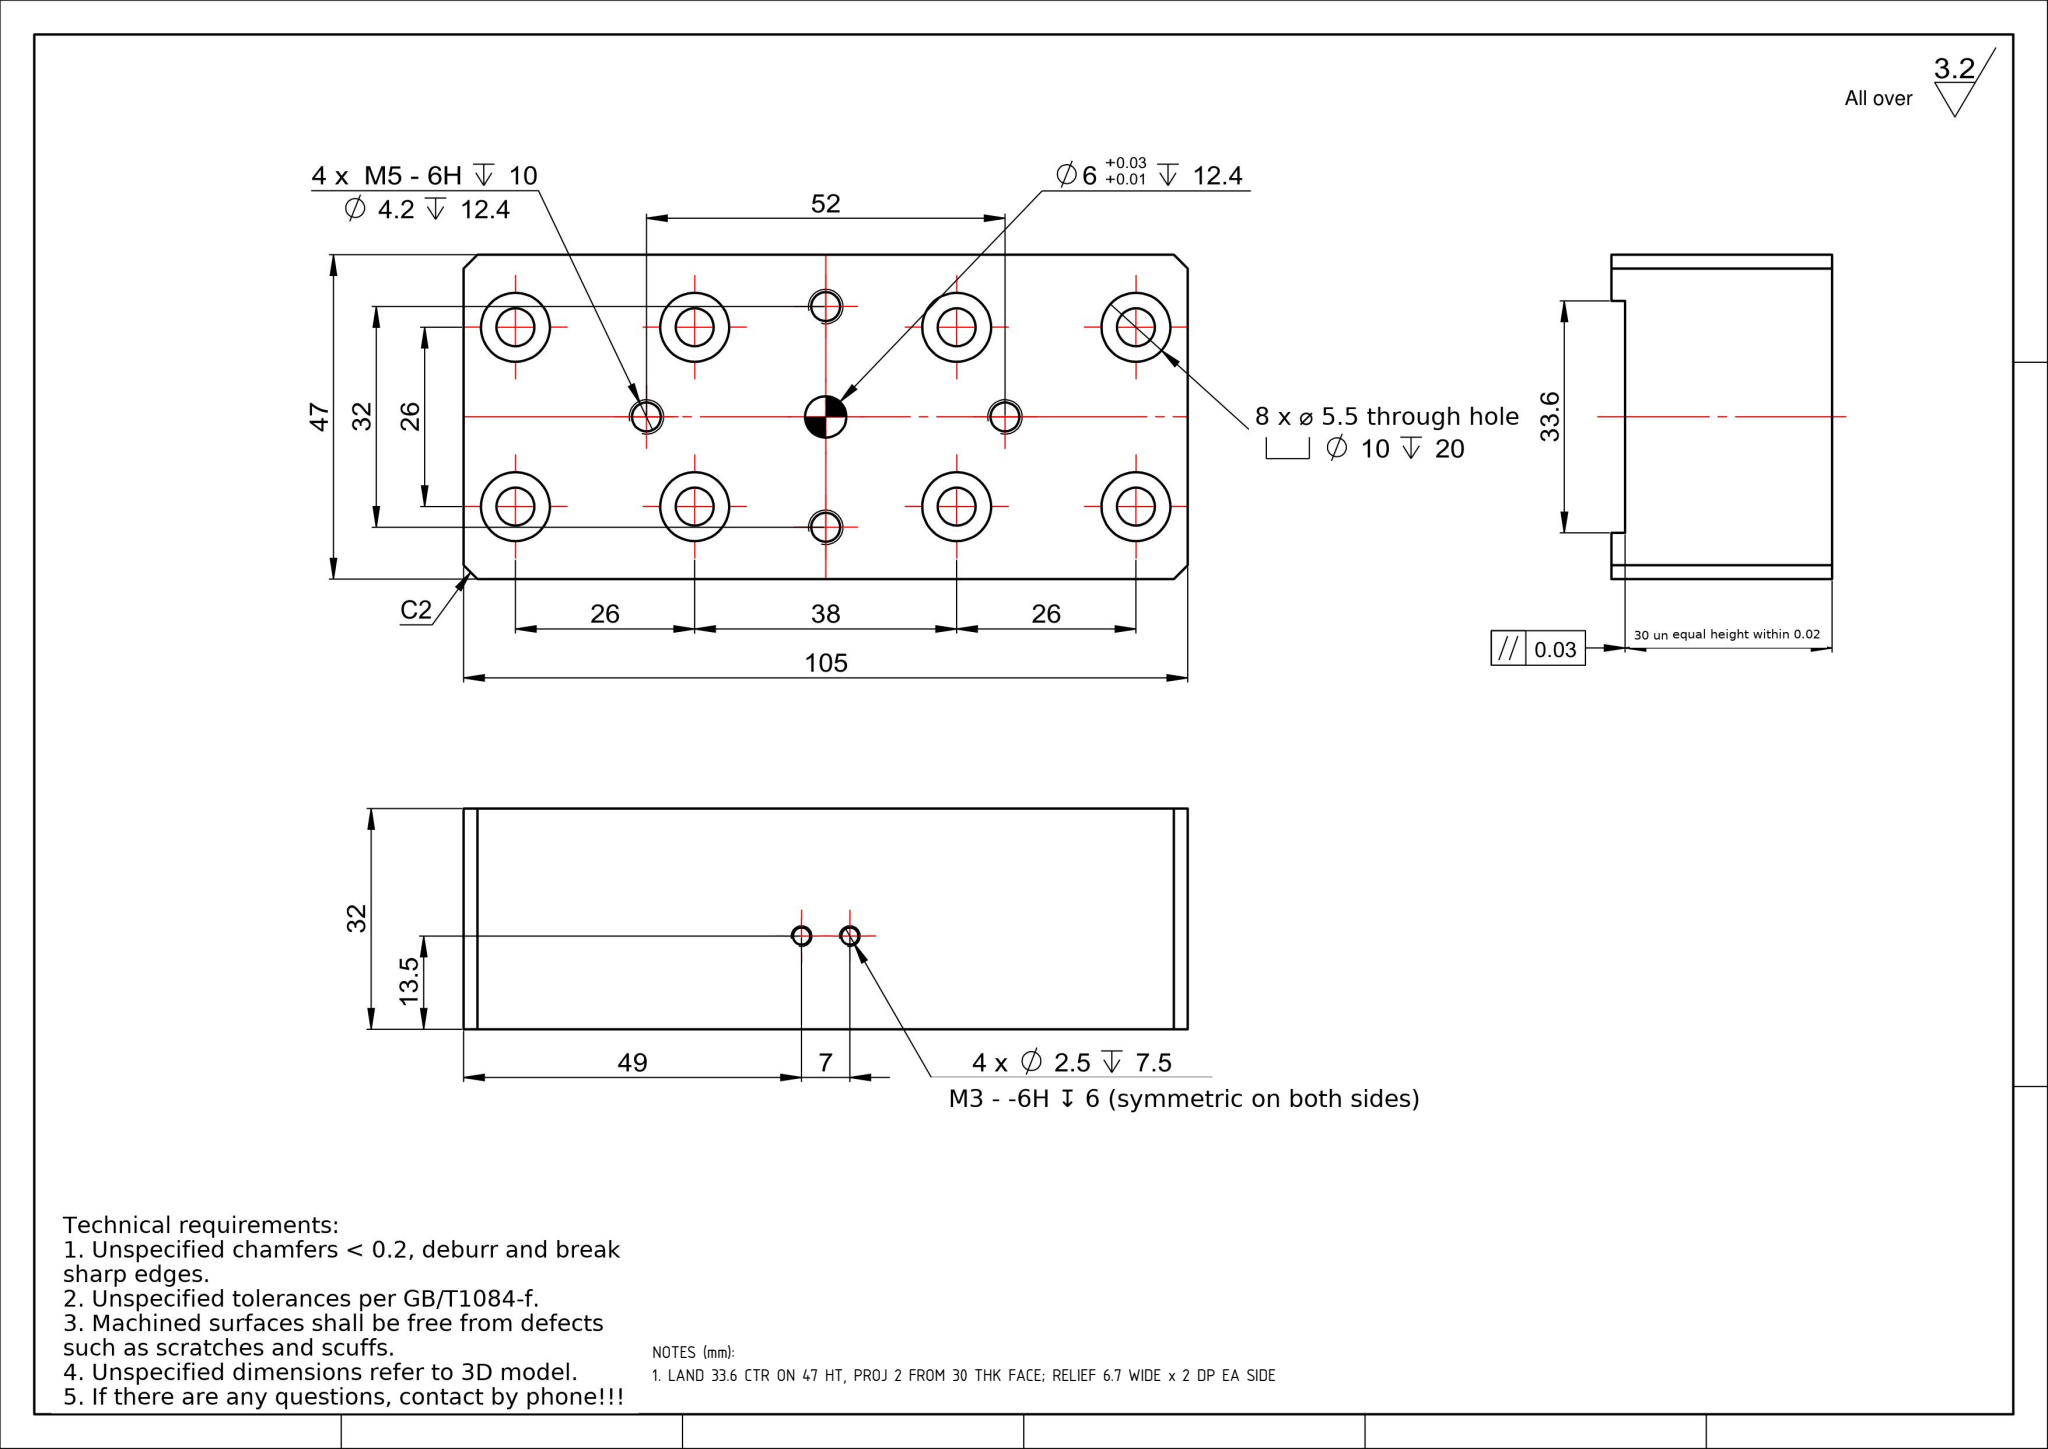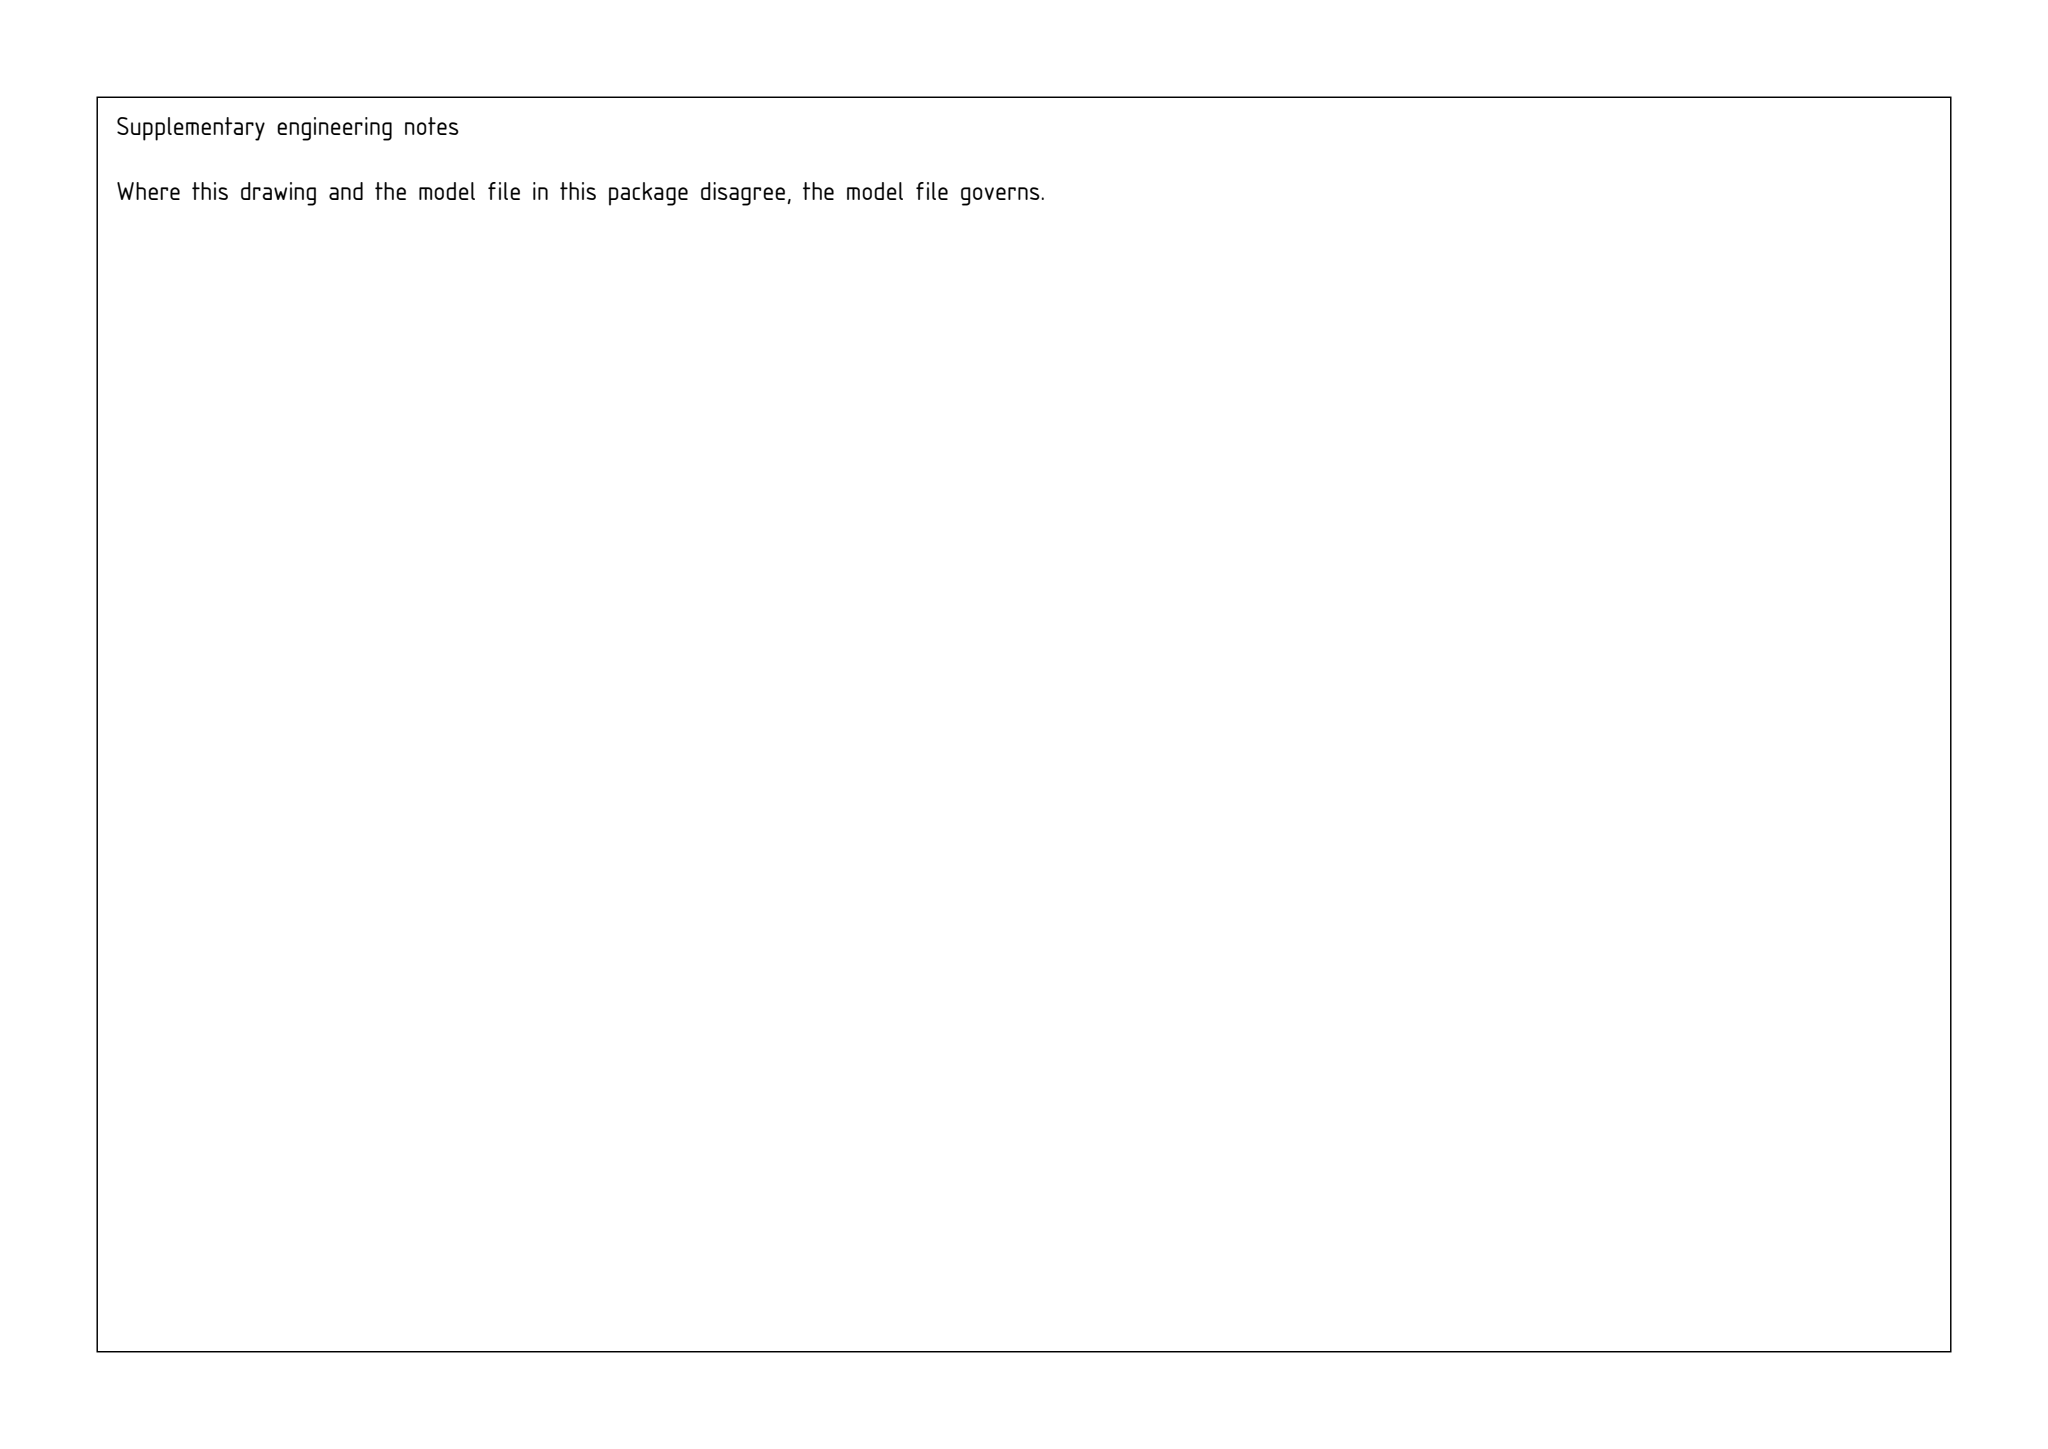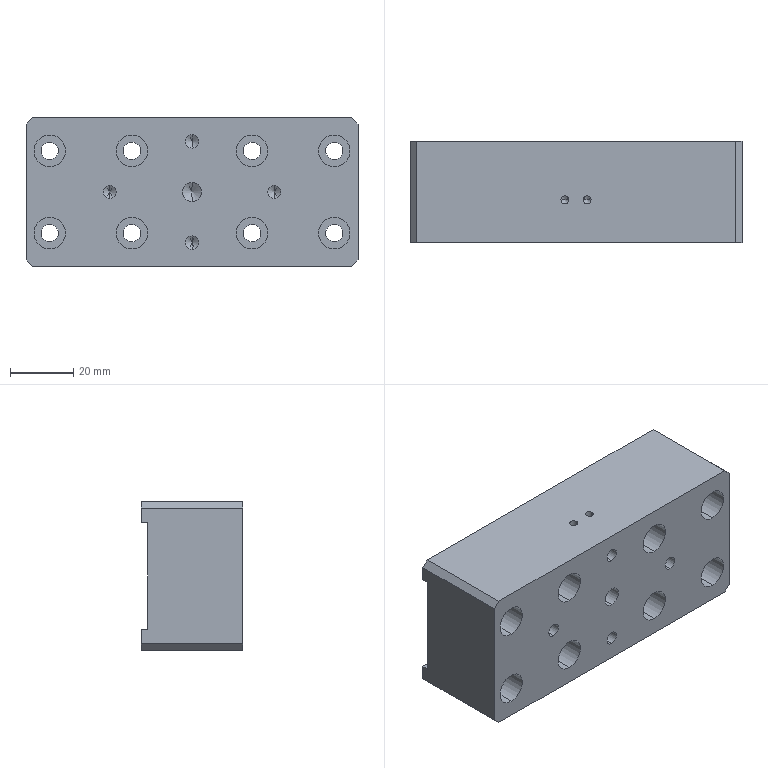Part | SolidWorks | mm | 1 solid | 90 faces | box 105 x 32 x 47 mm | volume 134911 mm3 | cylinder 50 | plane 22 | cone 18 | commonest cylinder face diameters 10 x16 5.5 x16 2.5 x8 4.2 x8 6 x2
Drawing notes:
LAND 33.6 CTR ON 47 HT, PROJ 2 FROM 30 THK FACE; RELIEF 6.7 WIDE x 2 DP EA SIDE | from the solid: z planes 0/6.7/40.3/47 give 33.6 land w/ 6.7 relief ea side; y=32 only over land, y=30 elsewhere (32-30=2); opposite face single plane y=0
build123d program:
from build123d import *

# Parameters (mm, degrees)
SKETCH1_W                                       = 105
SKETCH1_H                                       = 30
BOSS_EXTRUDE1_DEPTH                             = 47
SKETCH2_W                                       = 105
SKETCH2_H                                       = 6.7
BOSS_EXTRUDE2_DEPTH                             = 2
M5_TAPPED_HOLE1_D                               = 4.2
M5_TAPPED_HOLE1_DEPTH                           = 12.4
M5_TAPPED_HOLE1_TIP                             = 1.262
M3_TAPPED_HOLE1_AT_2_COUNT                      = 2
M3_TAPPED_HOLE1_AT_2_PITCH                      = 7
CHAMFER1_SIZE                                   = 2
SIZE_MM_DOWEL_PIN_HOLE_1_D                      = 6
SIZE_MM_DOWEL_PIN_HOLE_1_DEPTH                  = 12.4
SIZE_MM_DOWEL_PIN_HOLE_1_TIP                    = 1.803
M5_HEX_SOCKET_HEAD_CAP_SCREW_CBORE1_D           = 5.5
M5_HEX_SOCKET_HEAD_CAP_SCREW_CBORE1_CBORE_D     = 10
M5_HEX_SOCKET_HEAD_CAP_SCREW_CBORE1_CBORE_DEPTH = 20


with BuildPart() as part:
    # Sketch1 → Boss-Extrude1 (new body)
    with BuildSketch(Plane.XY):
        with Locations((52.5, 15)):
            Rectangle(SKETCH1_W, SKETCH1_H)
    extrude(amount=BOSS_EXTRUDE1_DEPTH)

    # Sketch2 → Boss-Extrude2 (add)
    with BuildSketch(Plane(origin=(0, 30, 0), x_dir=(1, 0, 0), z_dir=(0, 1, 0))):
        with Locations((52.5, -3.35)):
            Rectangle(SKETCH2_W, SKETCH2_H)
        with Locations((52.5, -43.65)):
            Rectangle(SKETCH2_W, SKETCH2_H)
    extrude(amount=BOSS_EXTRUDE2_DEPTH)

    # M5 Tapped Hole1
    with Locations(Plane(origin=(0, 0, 0), x_dir=(-1, 0, 0), z_dir=(0, -1, 0))):
        with Locations((-52.5, -7.5), (-52.5, -39.5), (-78.5, -23.5), (-26.5, -23.5)):
            Hole(M5_TAPPED_HOLE1_D / 2, depth=M5_TAPPED_HOLE1_DEPTH)
            with Locations((0, 0, -(M5_TAPPED_HOLE1_DEPTH + M5_TAPPED_HOLE1_TIP / 2))):  # 118° drill point
                Cone(0, M5_TAPPED_HOLE1_D / 2, M5_TAPPED_HOLE1_TIP, mode=Mode.SUBTRACT)

    # Sketch20 → M3 Tapped Hole1 (revolve, cut)
    with BuildSketch(Plane(origin=(49, 13.5, 0), x_dir=(0, 1, 0), z_dir=(1, 0, 0))):
        Polygon((0, 0), (0, 8.251), (1.25, 7.5), (1.25, 0), align=None)
    m3_tapped_hole1 = revolve(axis=Axis((49, 13.5, -6.35), (0, 0, 1)), mode=Mode.SUBTRACT)

    # M3 Tapped Hole1 at 2: M3 Tapped Hole1 ×2
    with Locations(*[(i * M3_TAPPED_HOLE1_AT_2_PITCH, 0, 0) for i in range(1, M3_TAPPED_HOLE1_AT_2_COUNT)]):
        add(m3_tapped_hole1, mode=Mode.SUBTRACT)

    # Mirror1: M3 Tapped Hole1 across plane
    add(m3_tapped_hole1.mirror(Plane(origin=(0, 0, 23.5), x_dir=(1, 0, 0), z_dir=(0, 0, -1))), mode=Mode.SUBTRACT)

    # Mirror1 copy 1 sketch → Mirror1 copy 1 (revolve, cut)
    with BuildSketch(Plane(origin=(56, 13.5, 47), x_dir=(0, 1, 0), z_dir=(1, 0, 0))):
        Polygon((0, 0), (0, -8.251), (1.25, -7.5), (1.25, 0), align=None)
    revolve(axis=Axis((56, 13.5, 53.35), (0, 0, 1)), mode=Mode.SUBTRACT)

    # Chamfer1
    chamfer1_edges = [part.edges().sort_by_distance(p)[0] for p in [
        (105, 16, 47),
        (0, 16, 47),
        (105, 16, 0),
        (0, 16, 0),
    ]]
    chamfer(chamfer1_edges, length=CHAMFER1_SIZE)

    # Size mm Dowel Pin Hole 1
    with Locations(Plane(origin=(0, 0, 0), x_dir=(-1, 0, 0), z_dir=(0, -1, 0))):
        with Locations((-52.5, -23.5)):
            Hole(SIZE_MM_DOWEL_PIN_HOLE_1_D / 2, depth=SIZE_MM_DOWEL_PIN_HOLE_1_DEPTH)
            with Locations((0, 0, -(SIZE_MM_DOWEL_PIN_HOLE_1_DEPTH + SIZE_MM_DOWEL_PIN_HOLE_1_TIP / 2))):  # 118° drill point
                Cone(0, SIZE_MM_DOWEL_PIN_HOLE_1_D / 2, SIZE_MM_DOWEL_PIN_HOLE_1_TIP, mode=Mode.SUBTRACT)

    # M5 Hex Socket Head Cap Screw CBORE1 (through all)
    with Locations(Plane(origin=(0, 0, 0), x_dir=(-1, 0, 0), z_dir=(0, -1, 0))):
        with Locations((-7.5, -10.5), (-33.5, -10.5), (-33.5, -36.5), (-7.5, -36.5), (-71.5, -36.5), (-97.5, -36.5), (-97.5, -10.5), (-71.5, -10.5)):
            CounterBoreHole(M5_HEX_SOCKET_HEAD_CAP_SCREW_CBORE1_D / 2, M5_HEX_SOCKET_HEAD_CAP_SCREW_CBORE1_CBORE_D / 2, M5_HEX_SOCKET_HEAD_CAP_SCREW_CBORE1_CBORE_DEPTH)


solid = part.part